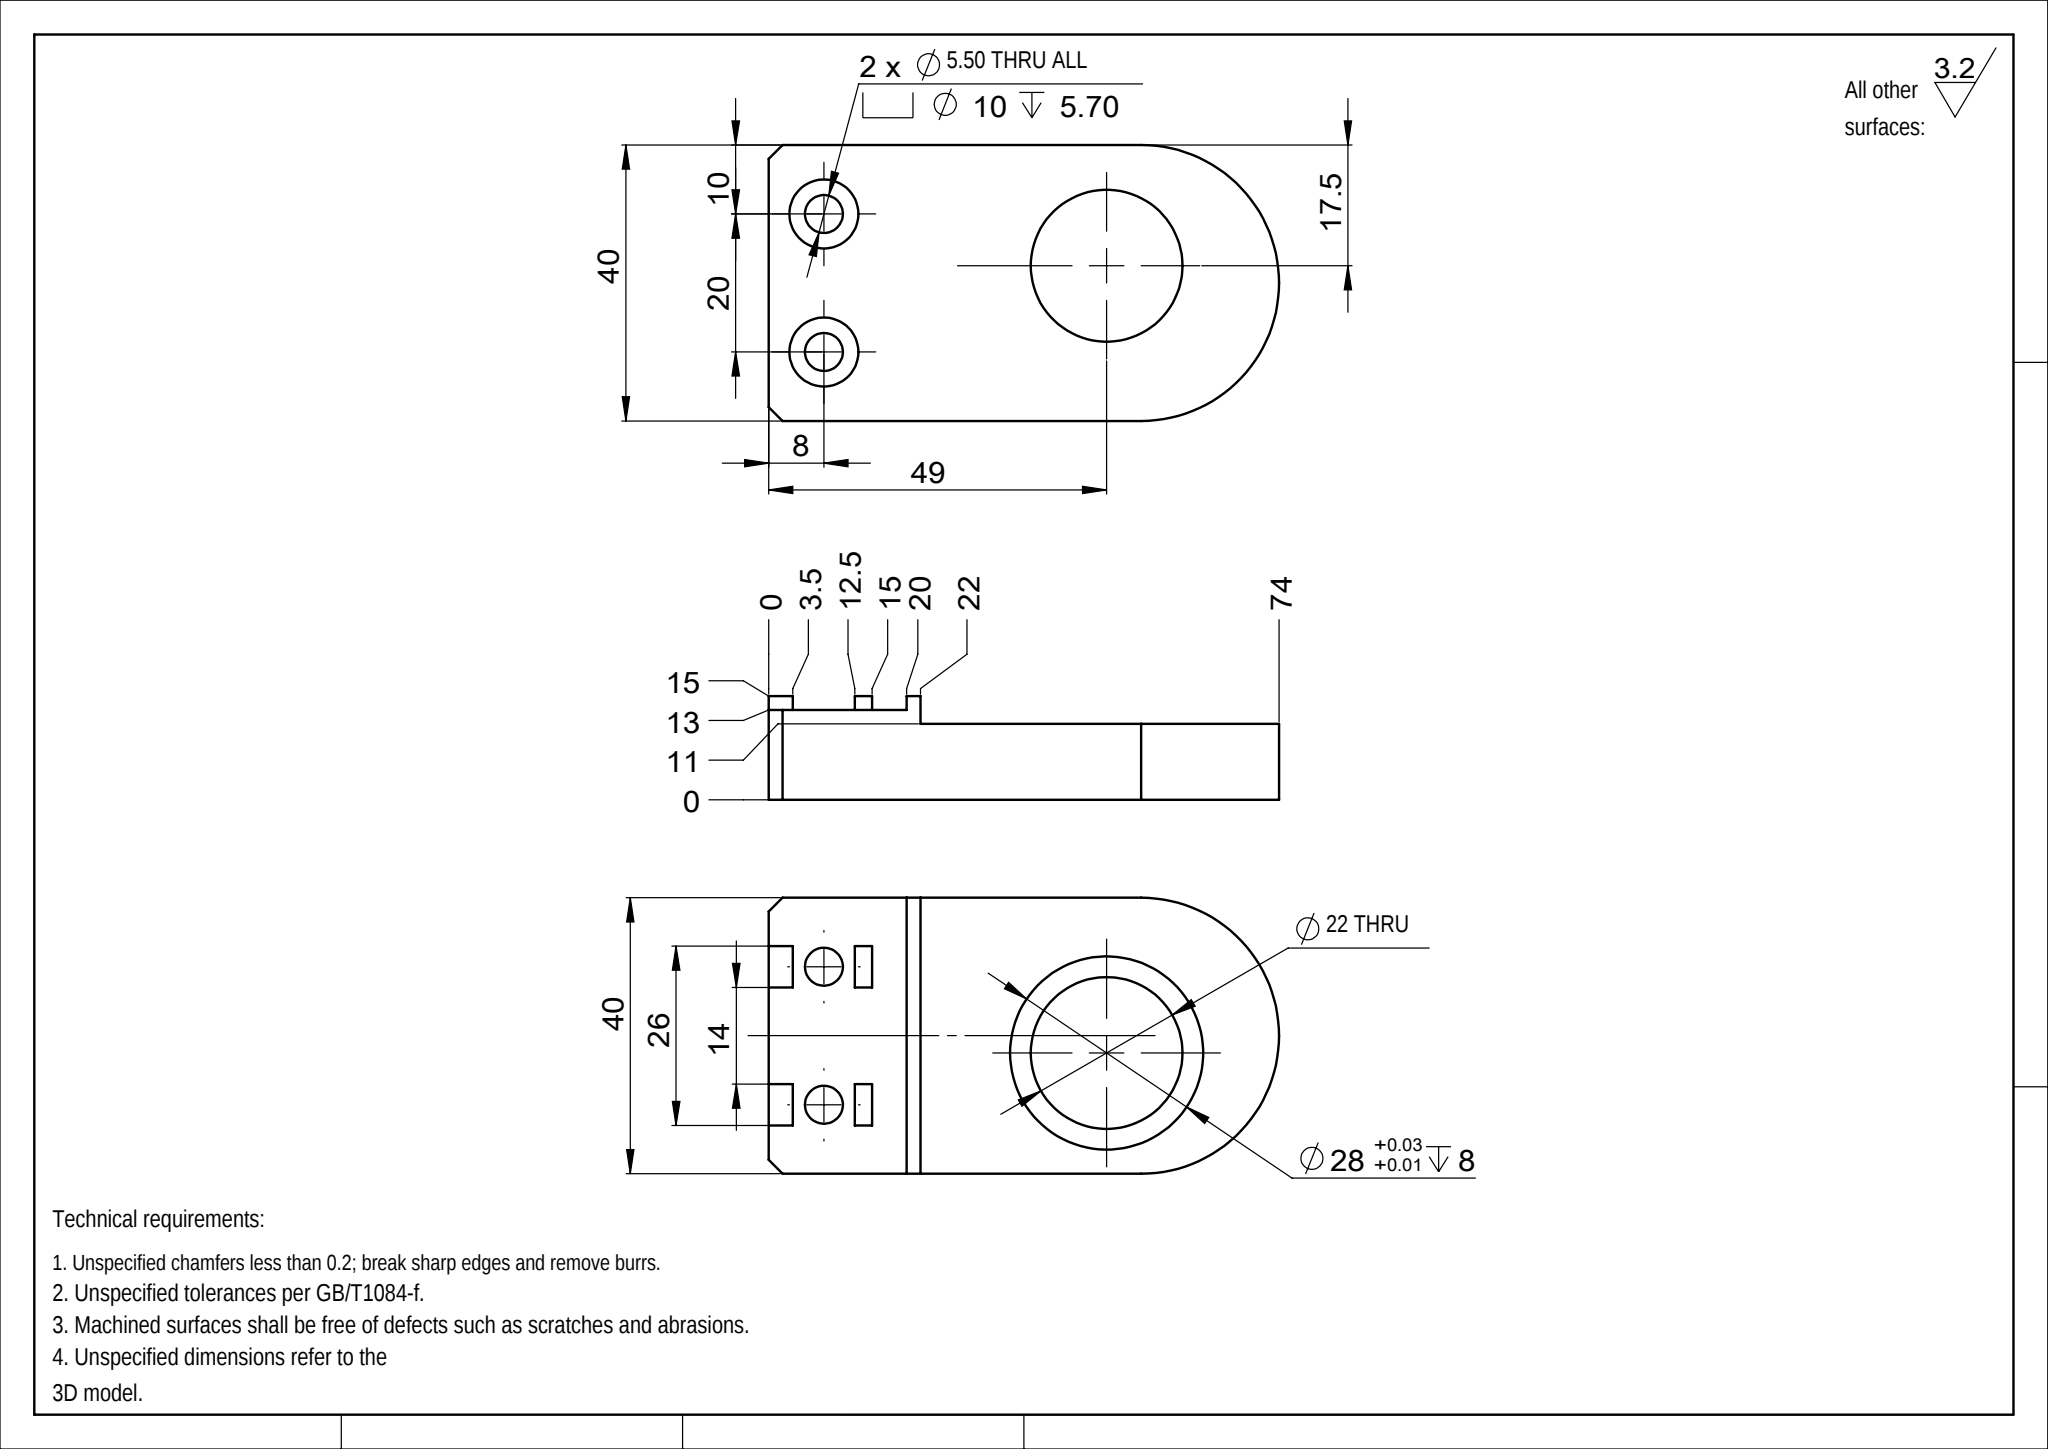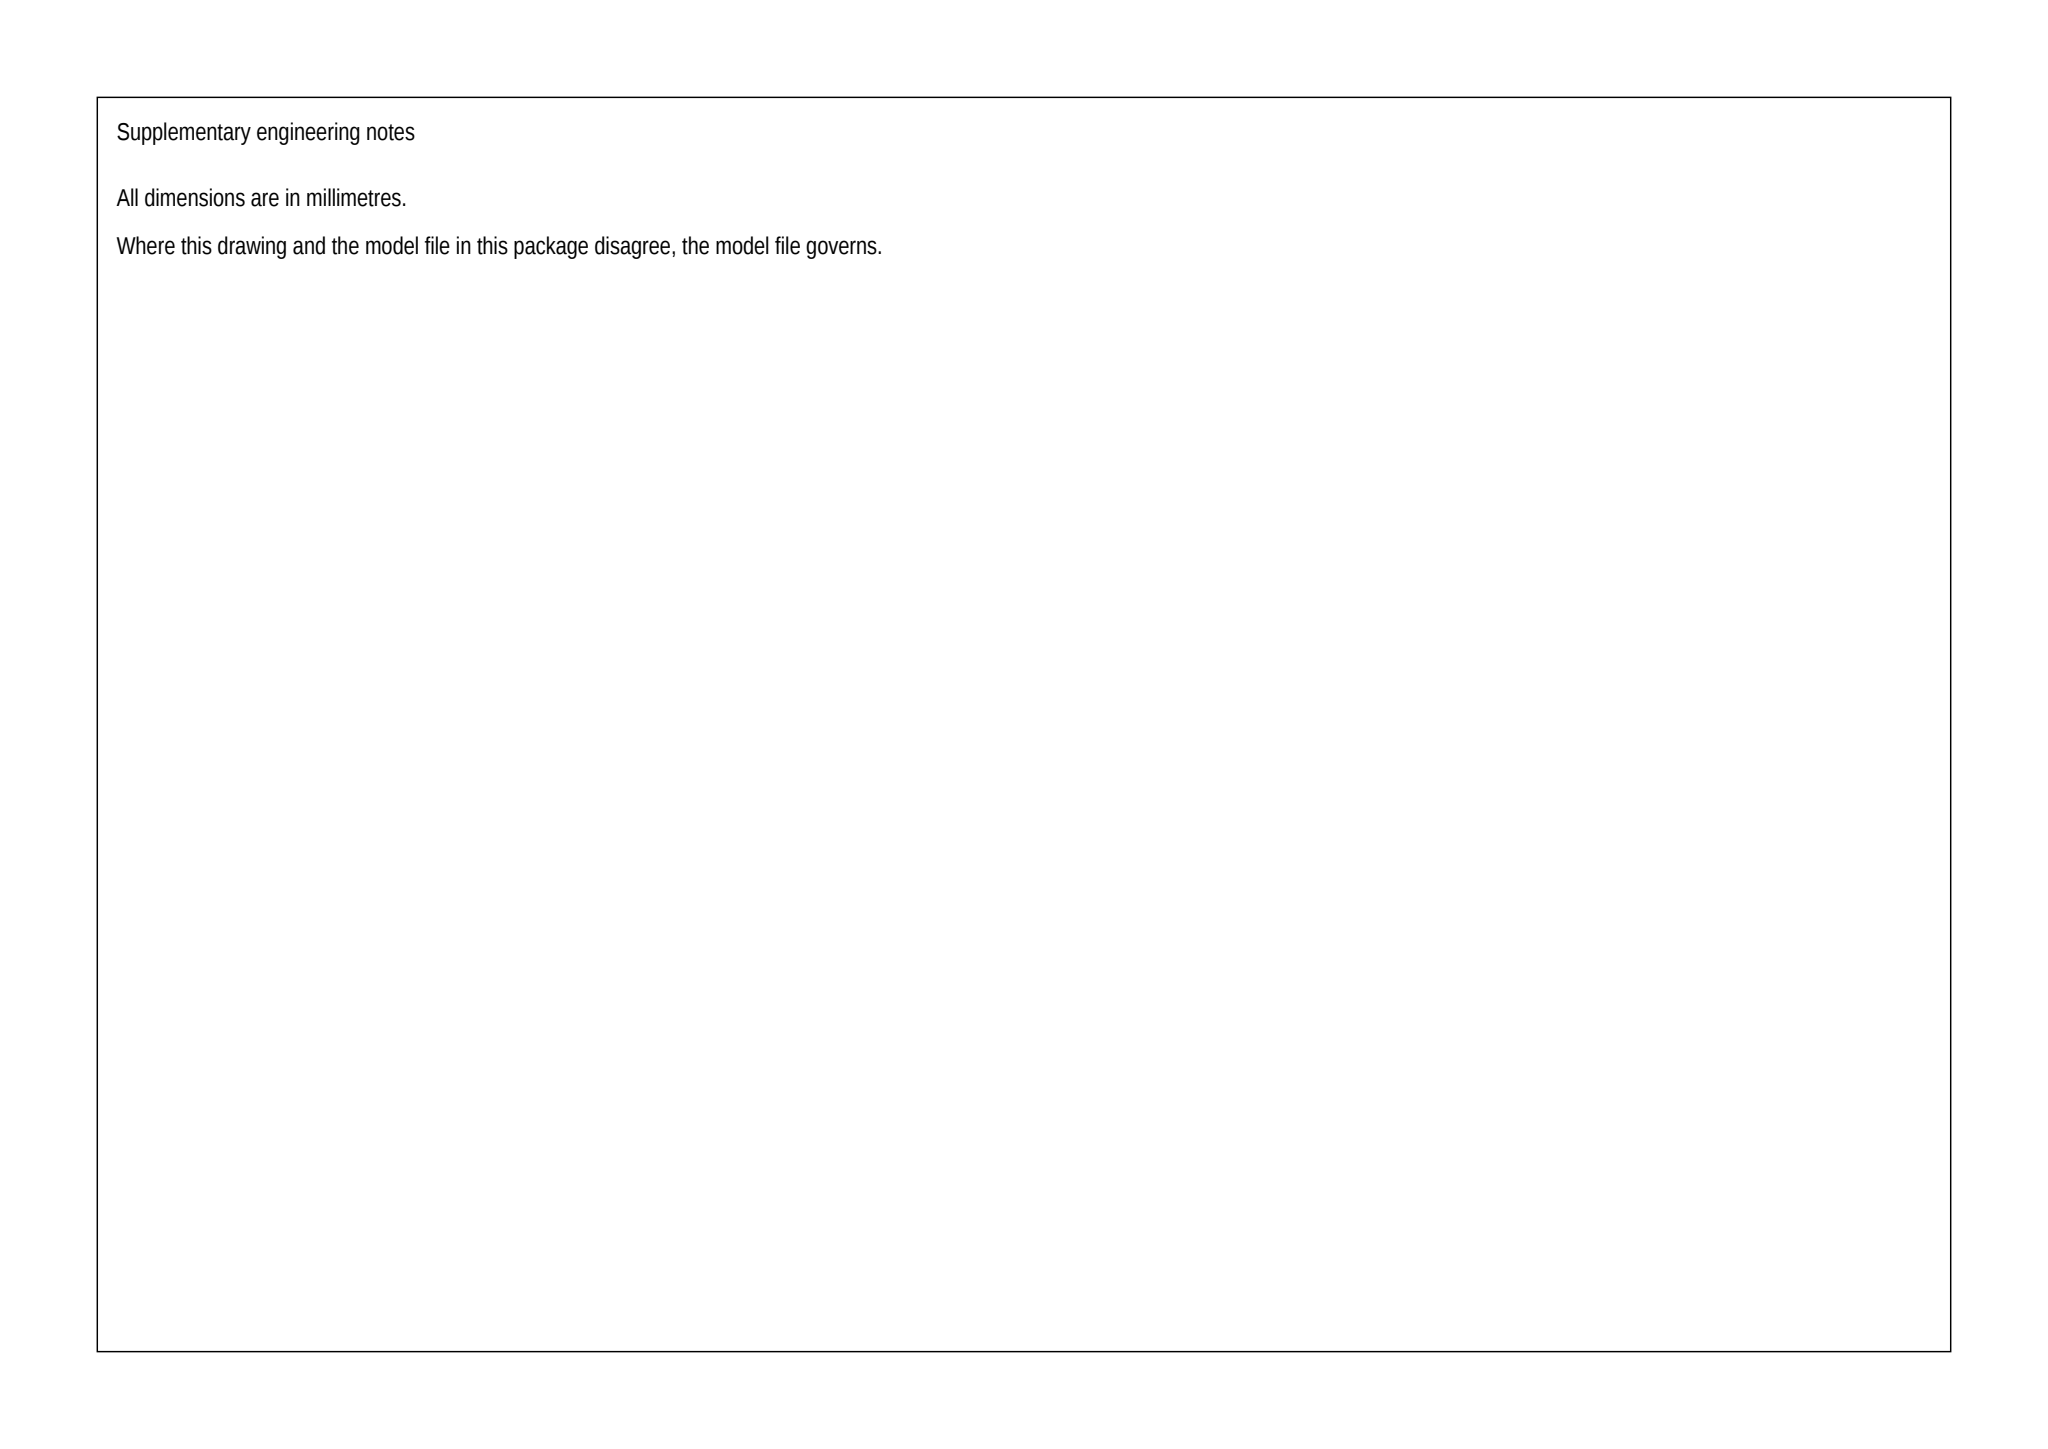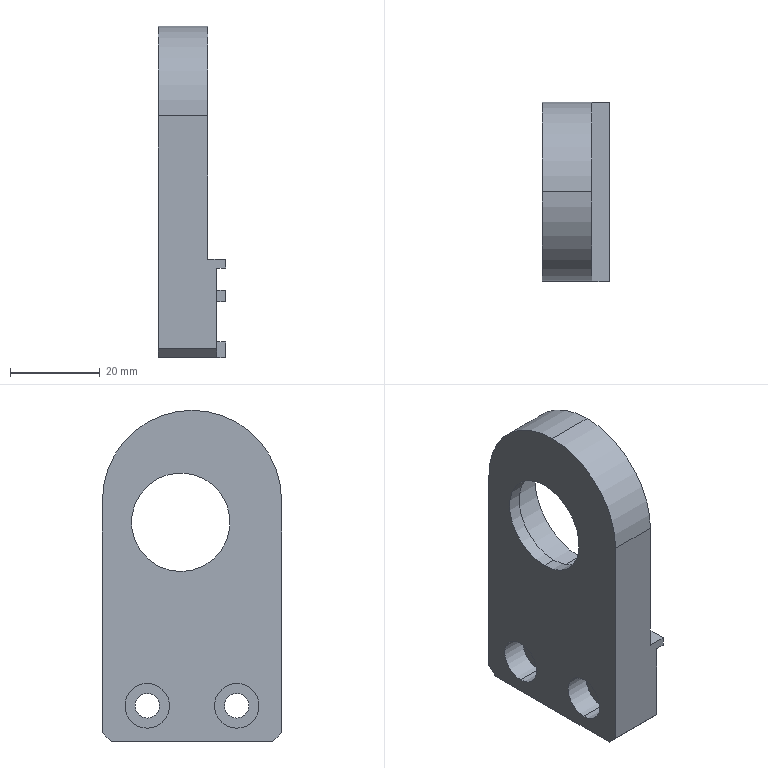Part | SolidWorks | mm | 1 solid | 46 faces | box 15 x 40 x 74 mm | volume 25375 mm3 | plane 32 | cylinder 14 | commonest cylinder face diameters 10 x4 5.5 x4 28 x2 22 x2 40 x2
Drawing notes:
4X PAD AT CBORES: 6 WIDE ON HOLE CL, 2 HIGH, 3.5 & 2.5 LG | from the solid: y-planes 7/13 and 27/33 = 6 wide ctr on hole axes y=10,30; z 0-3.5 and 12.5-15 = 3.5 & 2.5 lg; x=13 floor to x=15 pad top = 2 high; x=15 count 5
2X Ø5.50 THRU with Ø10 C'BORE 5.70 DEEP IS MACHINED FROM THE 0 FACE (THE FACE OPPOSITE THE 15 PAD FACE); C'BORE FLOOR LIES AT 5.70 FROM THAT 0 FACE. | from the solid: cylinders Ø10 axis x at y=10 and y=30, z=8, length 5.7 starting at x=0; axis_planes x=5.7 count 2 (c'bore floors)
2X CHAMFER 2 x 45 deg on the two long corners at the z=0 end of the plate (edges at y=0 and y=40), extending along x from x=0 to x=13 from the 0 face. | from the solid: inclined_planes: angle_to_xyz_axes [90,45,45], bbox_from [0,0,0] and [0,38,0], size [13,2,2]